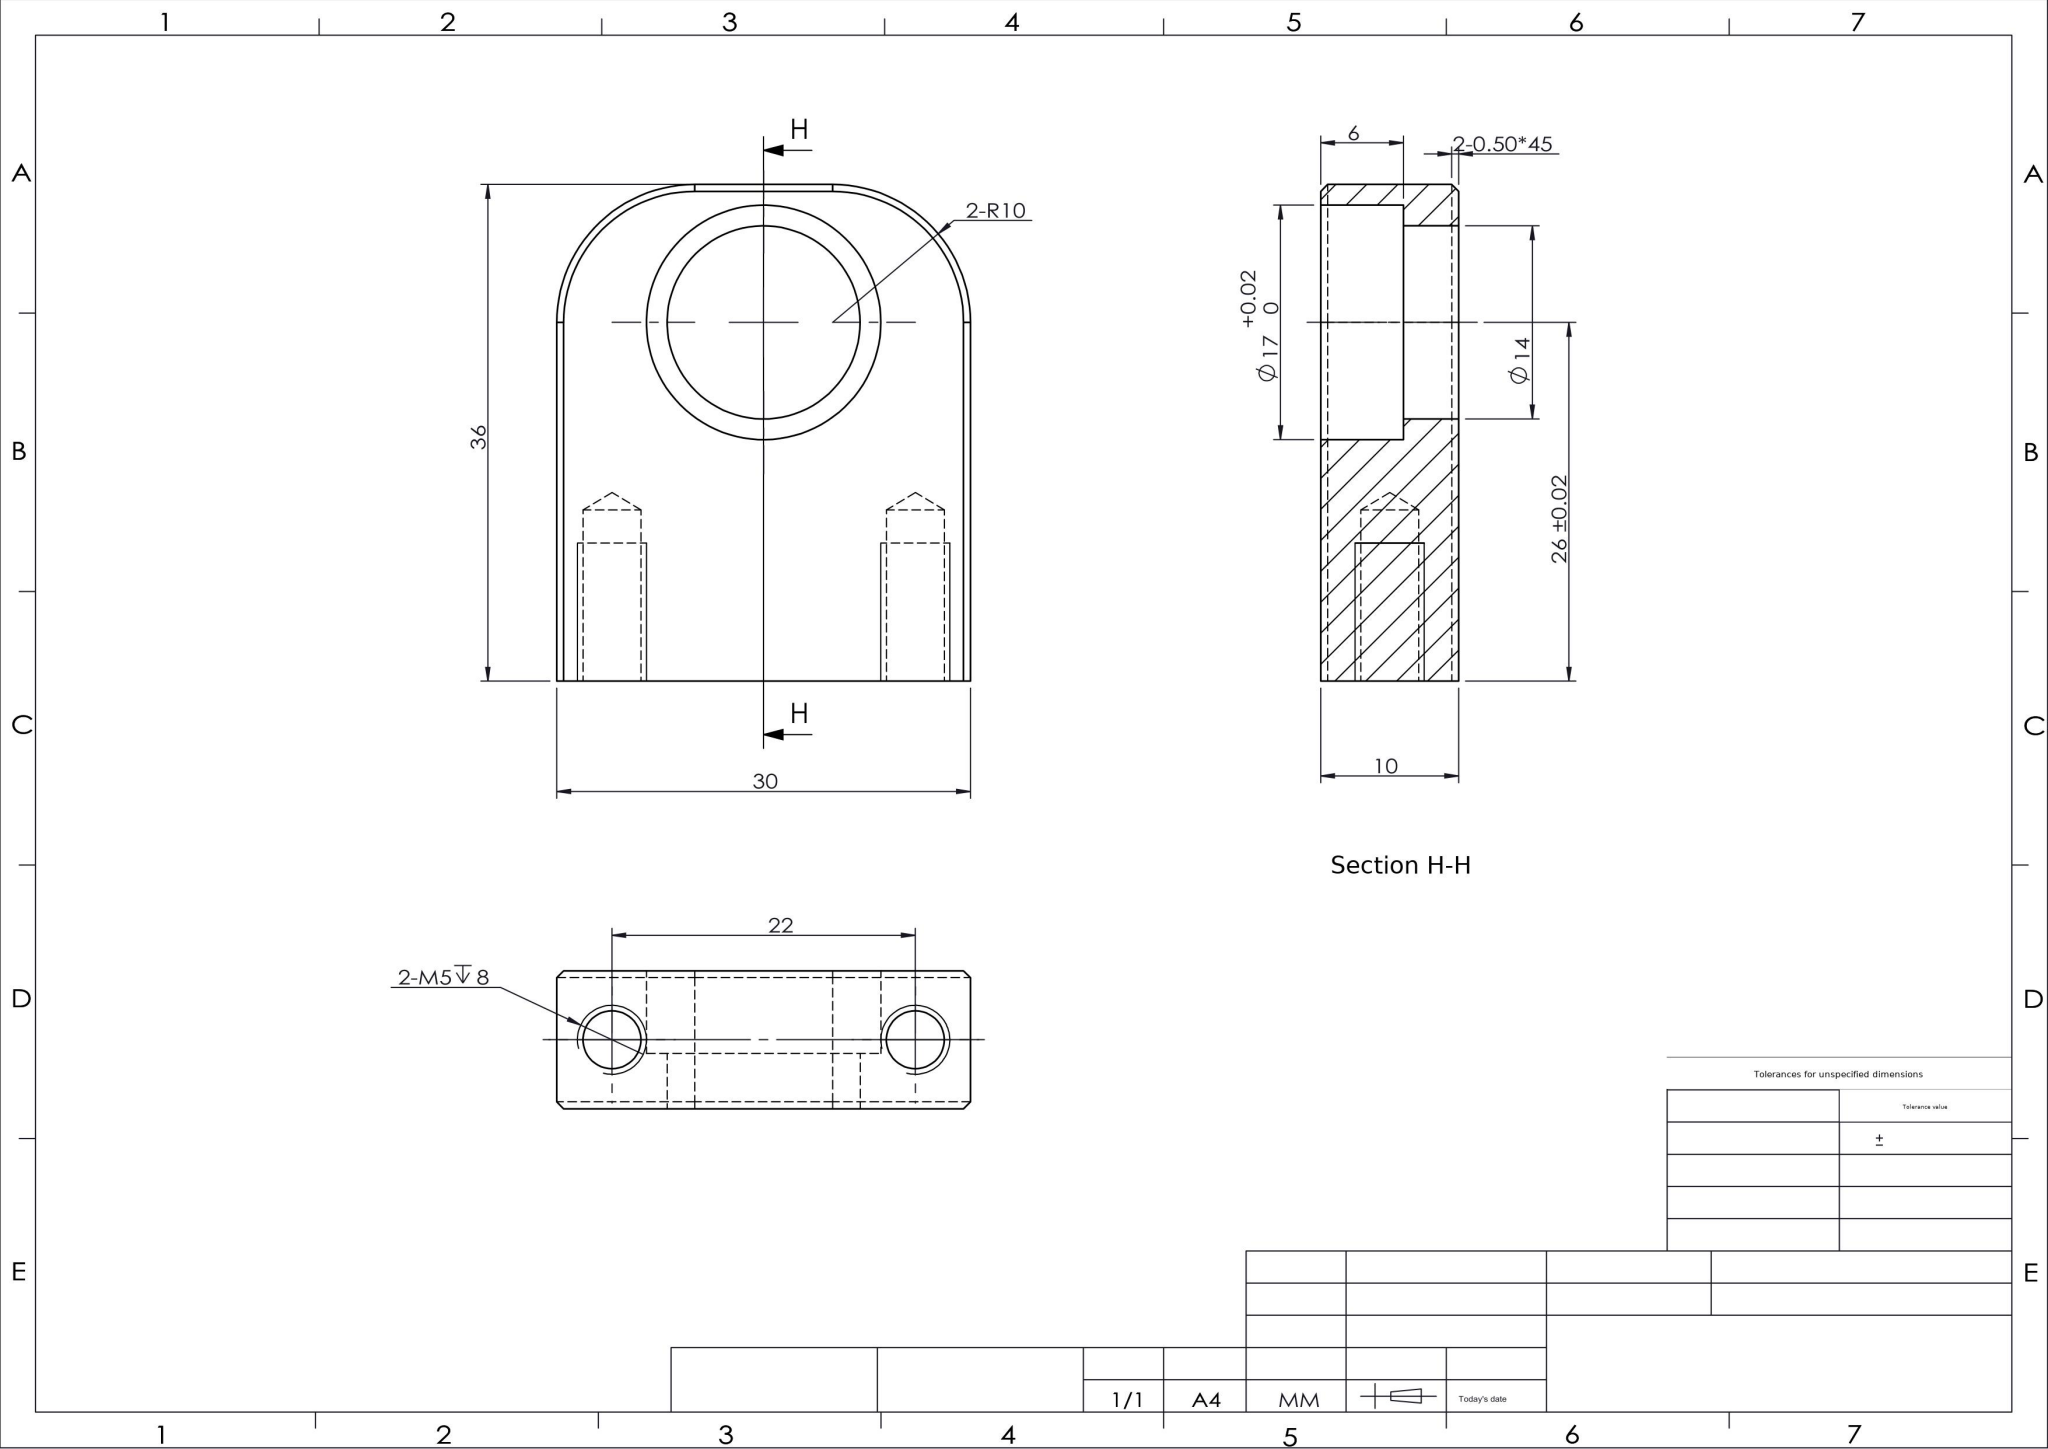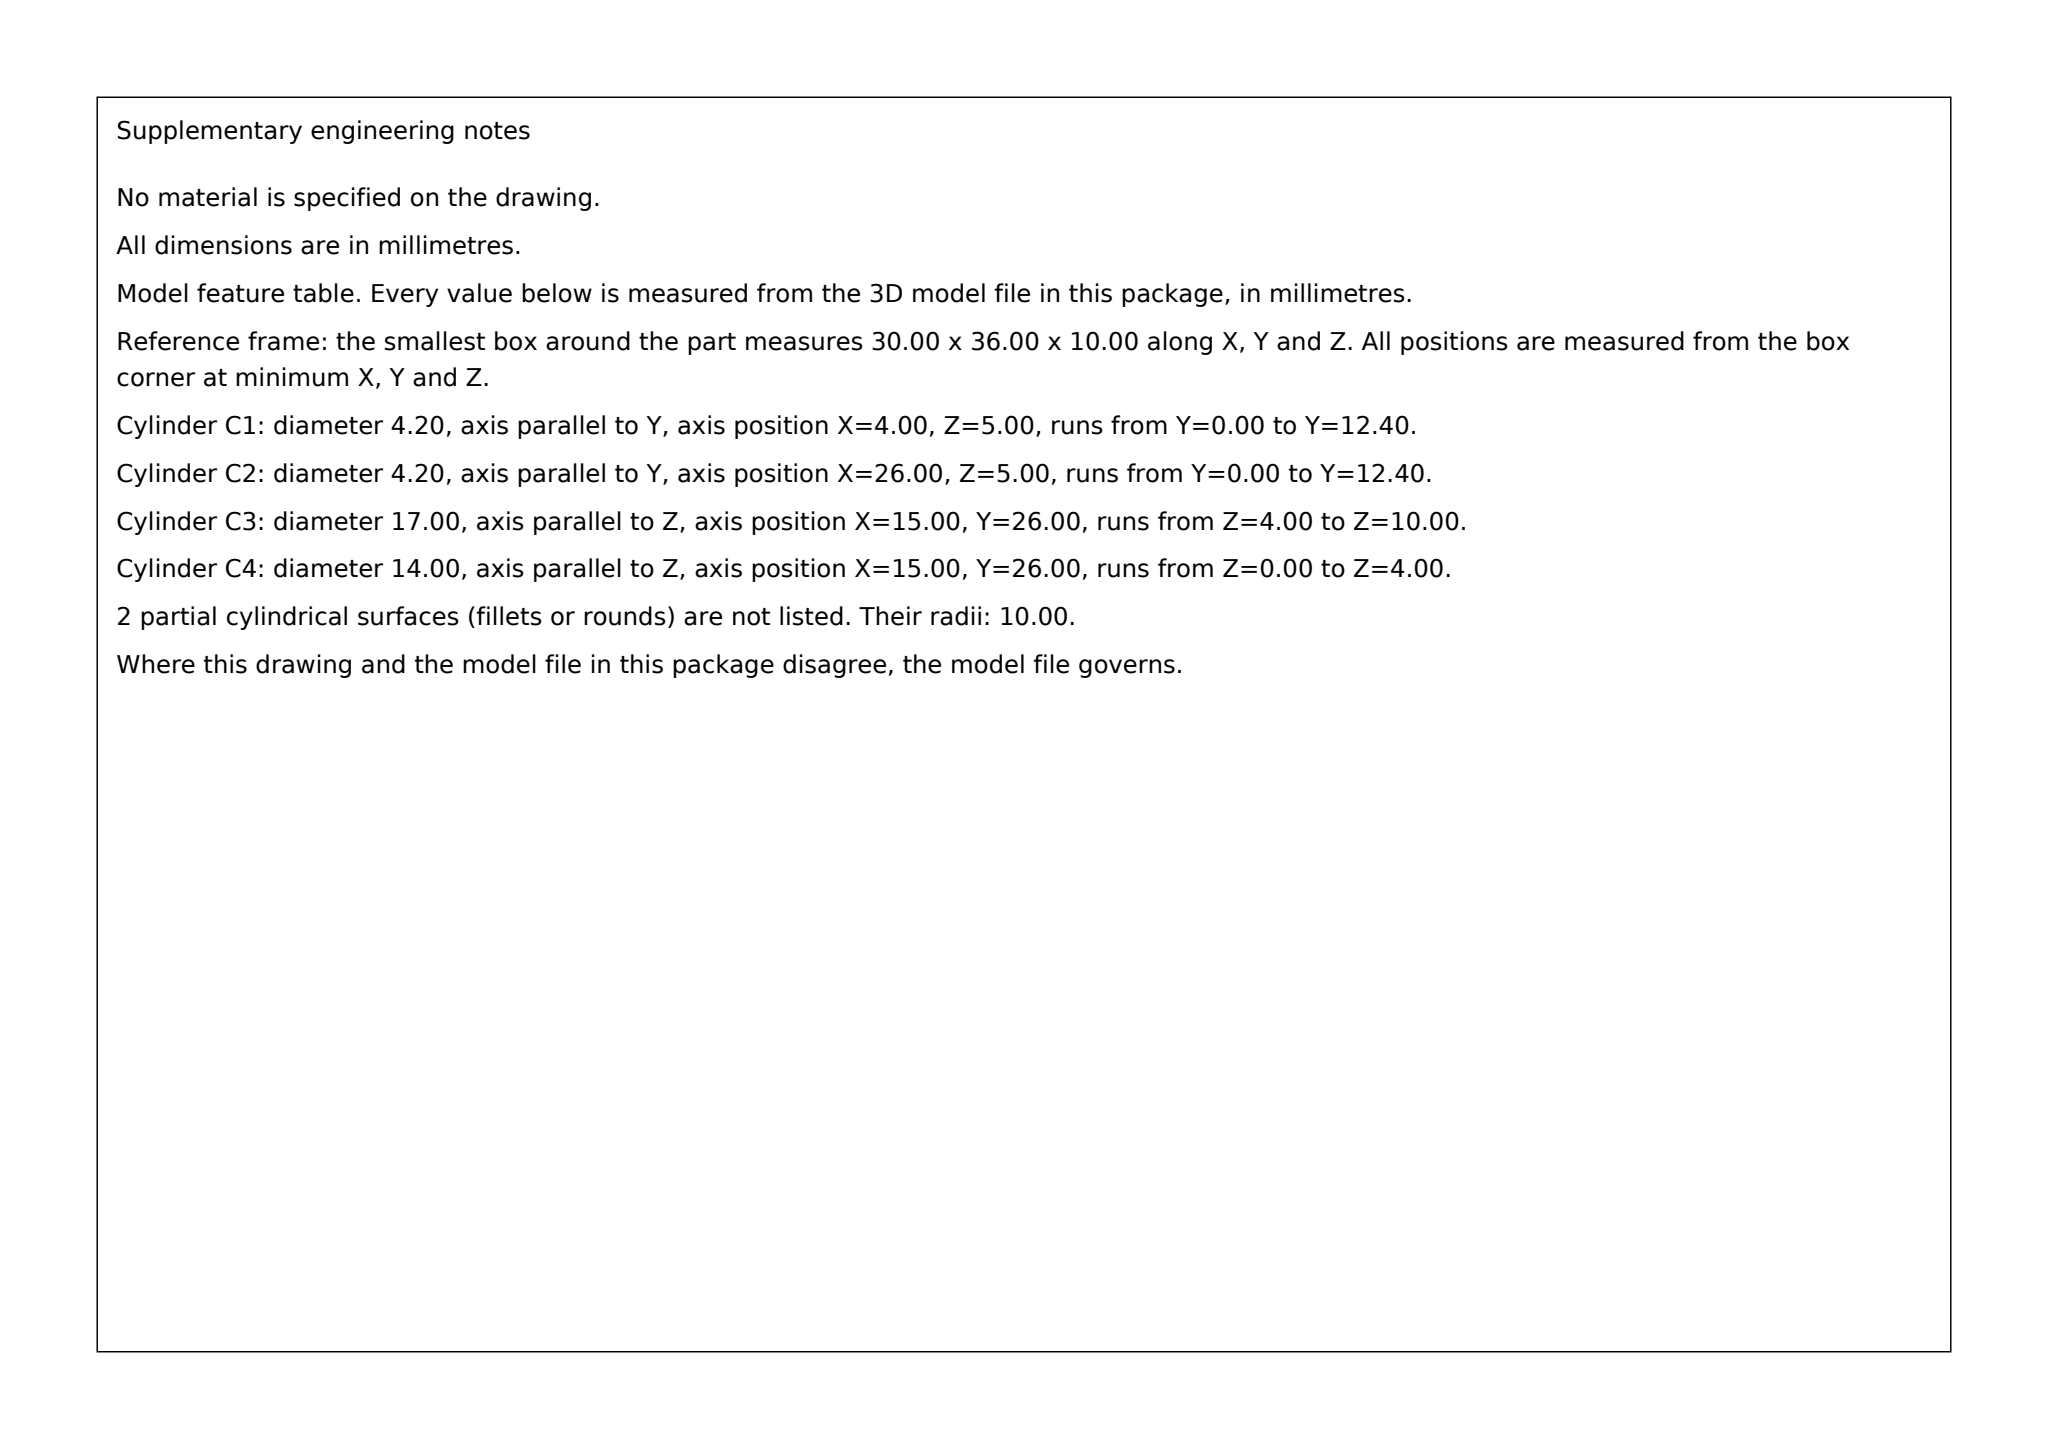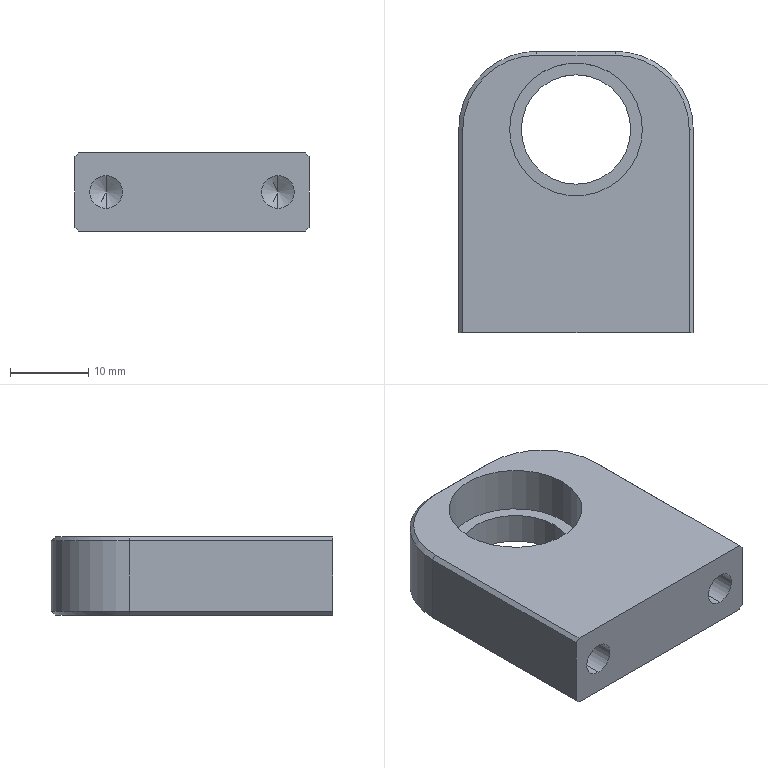Part | SolidWorks | mm | 1 solid | 31 faces | box 30 x 36 x 10 mm | volume 8015 mm3 | plane 13 | cylinder 10 | cone 8 | commonest cylinder face diameters 4.2 x4 17 x2 14 x2 20 x2
build123d program:
from build123d import *

# Parameters (mm, degrees)
SKETCH1_W             = 30
SKETCH1_H             = 36
BOSS_EXTRUDE1_DEPTH   = 10
SKETCH3_R             = 7
CUT_EXTRUDE2_DEPTH    = 48.917
FILLET1_R             = 10
SKETCH4_R             = 8.5
CUT_EXTRUDE3_DEPTH    = 6
M5_TAPPED_HOLE1_D     = 4.2
M5_TAPPED_HOLE1_DEPTH = 12.4
M5_TAPPED_HOLE1_TIP   = 1.262
CHAMFER1_SIZE         = 0.5


with BuildPart() as part:
    # Sketch1 → Boss-Extrude1 (new body)
    with BuildSketch(Plane.XY):
        with Locations((15, 18)):
            Rectangle(SKETCH1_W, SKETCH1_H)
    extrude(amount=BOSS_EXTRUDE1_DEPTH)

    # Sketch3 → Cut-Extrude2 (cut, through all)
    with BuildSketch(Plane.XY.offset(10)):
        with Locations((15, 26)):
            Circle(SKETCH3_R)
    extrude(amount=-CUT_EXTRUDE2_DEPTH, mode=Mode.SUBTRACT)

    # Fillet1
    fillet1_edges = [part.edges().sort_by_distance(p)[0] for p in [
        (0, 36, 5),
        (30, 36, 5),
    ]]
    fillet(fillet1_edges, radius=FILLET1_R)

    # Sketch4 → Cut-Extrude3 (cut)
    with BuildSketch(Plane.XY.offset(10)):
        with Locations((15, 26)):
            Circle(SKETCH4_R)
    extrude(amount=-CUT_EXTRUDE3_DEPTH, mode=Mode.SUBTRACT)

    # M5 Tapped Hole1
    with Locations(Plane(origin=(0, 0, 0), x_dir=(-1, 0, 0), z_dir=(0, -1, 0))):
        with Locations((-4, -5), (-26, -5)):
            Hole(M5_TAPPED_HOLE1_D / 2, depth=M5_TAPPED_HOLE1_DEPTH)
            with Locations((0, 0, -(M5_TAPPED_HOLE1_DEPTH + M5_TAPPED_HOLE1_TIP / 2))):  # 118° drill point
                Cone(0, M5_TAPPED_HOLE1_D / 2, M5_TAPPED_HOLE1_TIP, mode=Mode.SUBTRACT)

    # Chamfer1
    chamfer1_edges = [part.edges().sort_by_distance(p)[0] for p in [
        (30, 13, 10),
        (0, 13, 0),
        (0, 13, 10),
        (15, 36, 0),
        (27.071, 33.071, 0),
        (2.929, 33.071, 0),
        (15, 36, 10),
        (27.071, 33.071, 10),
        (2.929, 33.071, 10),
        (30, 13, 0),
    ]]
    chamfer(chamfer1_edges, length=CHAMFER1_SIZE)


solid = part.part